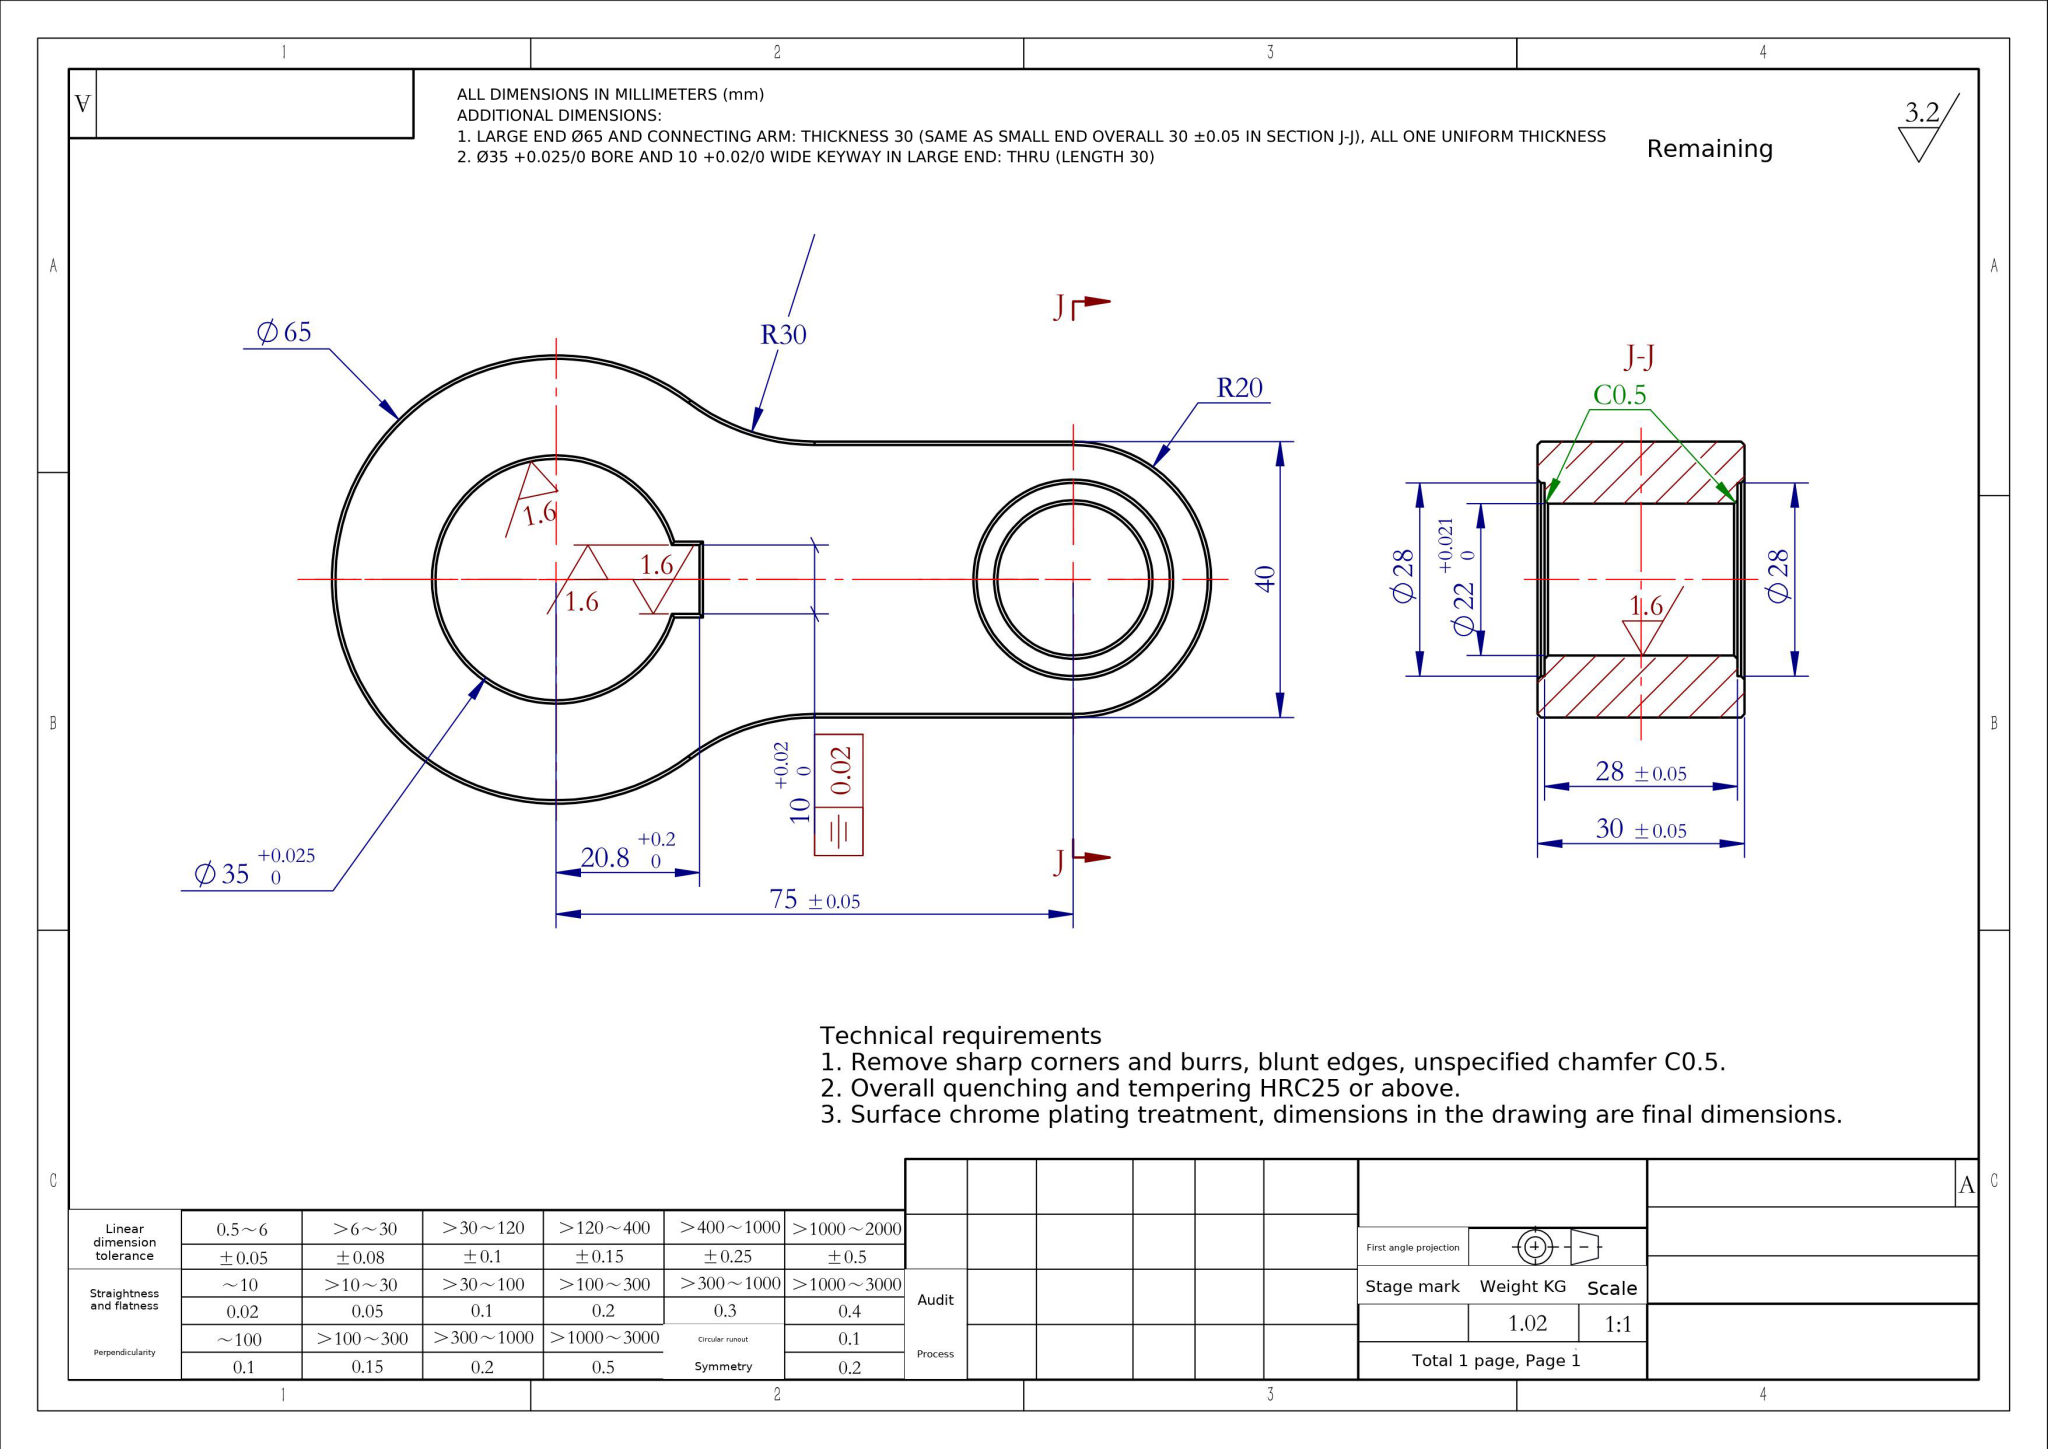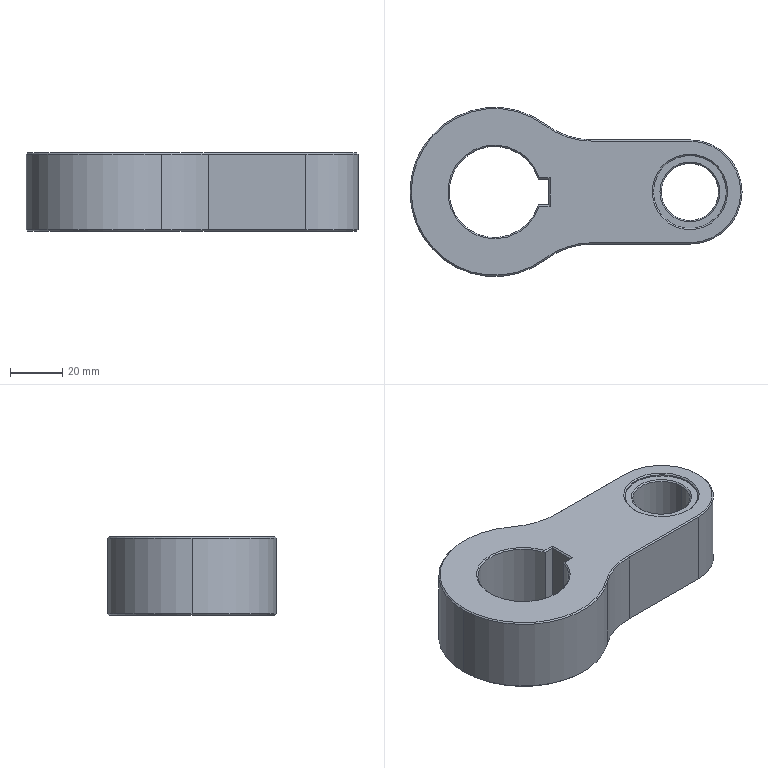Part | NX | mm | 1 solid | 55 faces | box 127.5 x 65 x 30 mm | volume 130940 mm3 | cone 22 | plane 19 | cylinder 14 | commonest cylinder face diameters 28 x4 35 x2 65 x2 22 x2 40 x2 60 x2